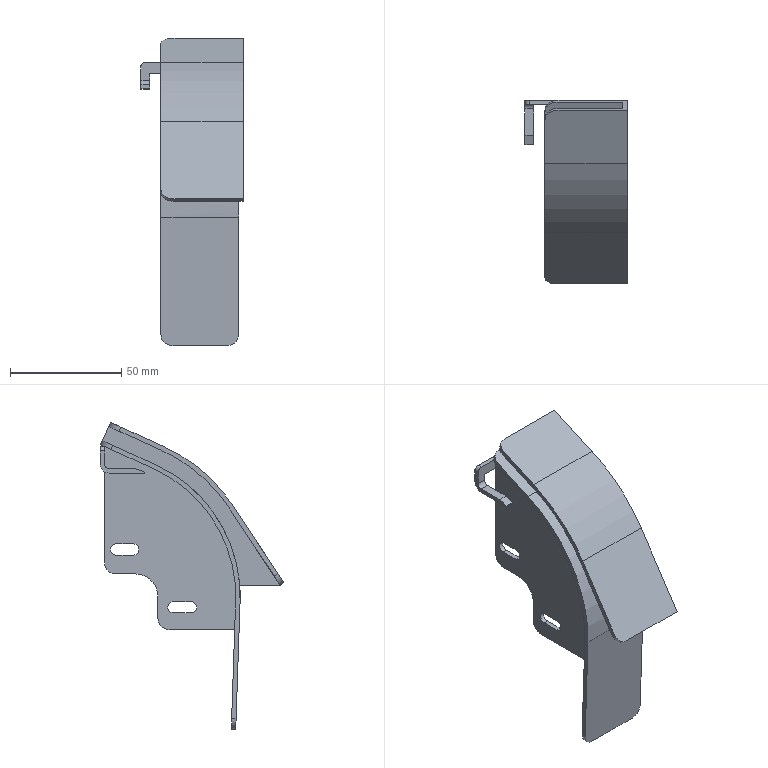Component | SolidWorks | ChainPartThreadGuide-1 | 3 solids | 60 faces | box 46 x 82.67 x 138.2 mm | volume 27719 mm3 | plane 40 | cylinder 20 | commonest cylinder face diameters 10 x7 5 x4 126 x2 4 x2 130 x1 144 x1 148 x1 8 x1
build123d program:
from build123d import *

# Parameters (mm, degrees)
EXTRUDE_THIN1_DEPTH = 17.5
BOSS_EXTRUDE1_DEPTH = 2
EXTRUDE_THIN2_START = -37
EXTRUDE_THIN2_DEPTH = 37
BOSS_EXTRUDE2_DEPTH = 2
CUT_EXTRUDE1_DEPTH  = 116.193
FILLET1_R           = 5
FILLET2_R           = 5
BOSS_EXTRUDE4_DEPTH = 2
SKETCH9_W           = 4
SKETCH9_H           = 20
BOSS_EXTRUDE5_DEPTH = 2
FILLET3_R           = 2
FILLET4_R           = 4
CHAMFER1_SIZE       = 1.5
CHAMFER1_SIZE2      = 4.121
FILLET5_R           = 2


with BuildPart() as part:
    # Sketch3 → Extrude-Thin1 (new, symmetric)
    with BuildSketch(Plane(origin=(0, 0, 0), x_dir=(0, 0, -1), z_dir=(1, 0, 0))):
        with BuildLine():
            Line((-75, -10), (-64.208, 13.823))
            ThreePointArc((-64.208, 13.823), (-39.292, 42.218), (-2.794, 51.963))
            Line((-2.794, 51.963), (55, 50))
            Line((55, 50), (54.932, 48.001))
            Line((54.932, 48.001), (-2.862, 49.964))
            ThreePointArc((-2.862, 49.964), (-38.237, 40.519), (-62.386, 12.997))
            Line((-62.386, 12.997), (-73.178, -10.825))
            Line((-73.178, -10.825), (-75, -10))
        make_face()
    extrude(amount=EXTRUDE_THIN1_DEPTH, both=True)

    # Sketch4 → Boss-Extrude1 (add)
    with BuildSketch(Plane.ZY.offset(17.5)):
        with BuildLine():
            Line((10, 49.801), (10, 70))
            Line((10, 70), (44.699, 47.066))
            ThreePointArc((44.699, 47.066), (59.786, 33.717), (70.584, 16.711))
            Line((70.584, 16.711), (81.376, -7.111))
            Line((81.376, -7.111), (73.178, -10.825))
            Line((73.178, -10.825), (62.386, 12.997))
            ThreePointArc((62.386, 12.997), (41.216, 38.55), (10, 49.801))
        make_face()
    extrude(amount=BOSS_EXTRUDE1_DEPTH)

    # Sketch5 → Extrude-Thin2 (add)
    with BuildSketch(Plane.ZY.offset(19.5).offset(EXTRUDE_THIN2_START)):
        with BuildLine():
            Line((81.376, -7.111), (70.584, 16.711))
            ThreePointArc((70.584, 16.711), (59.786, 33.717), (44.699, 47.066))
            Line((44.699, 47.066), (10, 70))
            Line((10, 70), (11.103, 71.669))
            Line((11.103, 71.669), (45.802, 48.735))
            ThreePointArc((45.802, 48.735), (61.308, 35.015), (72.406, 17.537))
            Line((72.406, 17.537), (83.198, -6.286))
            Line((83.198, -6.286), (81.376, -7.111))
        make_face()
    extrude(amount=EXTRUDE_THIN2_DEPTH)

    # Fillet1
    fillet1_edges = [part.edges().sort_by_distance(p)[0] for p in [
        (17.5, -6.699, 82.287),
        (17.5, -10.413, 74.089),
        (17.5, 70.834, 10.551),
        (-17.5, 49.001, -54.966),
        (17.5, 49.001, -54.966),
    ]]
    fillet(fillet1_edges, radius=FILLET1_R)


with BuildPart() as body_2:
    # Sketch6 → Boss-Extrude2 (new body)
    with BuildSketch(Plane(origin=(15.3, 0, 0), x_dir=(0, 0, -1), z_dir=(1, 0, 0))):
        with BuildLine():
            Line((-2.862, 49.964), (10, 49.527))
            Line((10, 49.527), (10, 15))
            Line((10, 15), (-5, 15))
            ThreePointArc((-5, 15), (-12.071, 12.071), (-15, 5))
            Line((-15, 5), (-15, -9))
            Line((-15, -9), (-72.351, -9))
            Line((-72.351, -9), (-62.386, 12.997))
            ThreePointArc((-62.386, 12.997), (-38.237, 40.519), (-2.862, 49.964))
        make_face()
    extrude(amount=-BOSS_EXTRUDE2_DEPTH)

    # Sketch7 → Cut-Extrude1 (cut, through all)
    with BuildSketch(Plane(origin=(15.3, 0, 0), x_dir=(0, 0, -1), z_dir=(1, 0, 0))):
        with BuildLine():
            Line((2.5, 30), (2.5, 22))
            ThreePointArc((2.5, 22), (0, 19.5), (-2.5, 22))
            Line((-2.5, 22), (-2.5, 30))
            ThreePointArc((-2.5, 30), (0, 32.5), (2.5, 30))
        make_face()
        with BuildLine():
            Line((-23.5, 4), (-23.5, -4))
            ThreePointArc((-23.5, -4), (-26, -6.5), (-28.5, -4))
            Line((-28.5, -4), (-28.5, 4))
            ThreePointArc((-28.5, 4), (-26, 6.5), (-23.5, 4))
        make_face()
    extrude(amount=-CUT_EXTRUDE1_DEPTH, mode=Mode.SUBTRACT)

    # Fillet2
    fillet2_edges = [body_2.edges().sort_by_distance(p)[0] for p in [
        (14.3, 15, -10),
        (14.3, -9, 15),
    ]]
    fillet(fillet2_edges, radius=FILLET2_R)


with BuildPart() as body_3:
    # Sketch8 → Boss-Extrude4 (new body)
    with BuildSketch(Plane.XZ.offset(9)):
        Polygon((6.5, 72.351), (26.5, 72.351), (26.5, 60.351), (22.5, 60.351), (22.5, 67.351), (6.5, 67.351), align=None)
    extrude(amount=BOSS_EXTRUDE4_DEPTH)

    # Sketch9 → Boss-Extrude5 (add)
    with BuildSketch(Plane(origin=(0, 0, 60.351), x_dir=(-1, 0, 0), z_dir=(0, 0, -1))):
        with Locations((-24.5, -1)):
            Rectangle(SKETCH9_W, SKETCH9_H)
    extrude(amount=-BOSS_EXTRUDE5_DEPTH)

    # Fillet3
    fillet3_edges = [body_3.edges().sort_by_distance(p)[0] for p in [
        (24.5, -9, 62.351),
    ]]
    fillet(fillet3_edges, radius=FILLET3_R)

    # Fillet4
    fillet4_edges = [body_3.edges().sort_by_distance(p)[0] for p in [
        (24.5, -11, 60.351),
    ]]
    fillet(fillet4_edges, radius=FILLET4_R)

    # Chamfer1
    chamfer1_edges = [body_3.edges().sort_by_distance(p)[0] for p in [
        (24.5, 9, 62.351),
    ]]
    chamfer1_side = [body_3.faces().sort_by_distance(p)[0] for p in [
        (24.5, 9, 61.351),
    ]]
    chamfer(chamfer1_edges, length=CHAMFER1_SIZE, length2=CHAMFER1_SIZE2, reference=chamfer1_side[0])

    # Fillet5
    fillet5_edges = [body_3.edges().sort_by_distance(p)[0] for p in [
        (26.5, -10, 72.351),
    ]]
    fillet(fillet5_edges, radius=FILLET5_R)


solid = Compound([part.part, body_2.part, body_3.part])

# Placed as in the assembly
solid = solid.moved(Location((160.737, -2.563, -35.304), (0, 0, 180)))